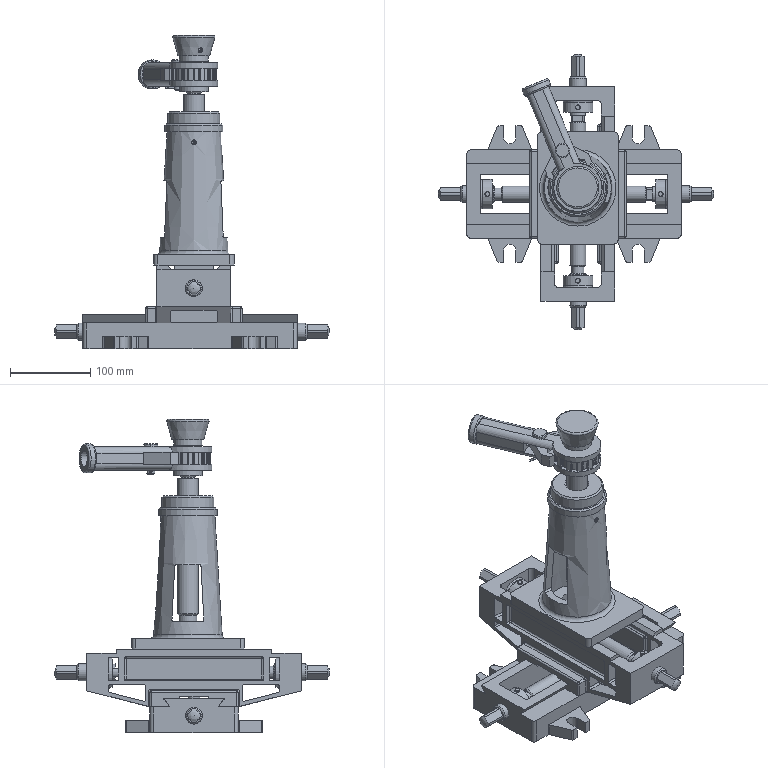Assembly | NX | mm | 32 component files | 32 solids | 906 faces | box 343 x 343 x 389.97 mm | volume 2573782 mm3 | cylinder 385 | plane 363 | cone 66 | torus 45 | sphere 40 | spline 7 | commonest cylinder face diameters 4 x153 2 x47 6 x35 10 x17 17 x16 56 x12 50 x12 21 x12
Bill of materials:
unnamed part 1 | 4 |  | Plain solid cylindrical pin with a chamfer at both ends.
unnamed part 2 | 1 |  | Prismatic block with a cross-section shaped like a rectangle with four chamfered corners (an elongated octagon). A single round through-bore runs the full length.
unnamed part 3 | 4 |  | Thick cylindrical ring or collar with a large central bore and one small radial cross-hole through the wall.
unnamed part 4 | 2 |  | Stepped cylindrical pin. A large-diameter body with a straight slot across its end steps down through a conical shoulder to a smaller-diameter spigot.
unnamed part 5 | 1 |  | Flanged cylindrical bushing with a through-bore, a chamfered flange and end, and one small radial hole in the shank.
unnamed part 6 | 2 |  | Long stepped shaft. It has a flatted tang at each end with a cross-hole, a raised collar section, a narrow necked groove, and a long main cylindrical section.
unnamed part 7 | 1 |  | Hollow, slightly tapered tubular post standing on a rectangular base plate with rounded corners. The tube wall has a rectangular side window. Two lugs project below the base, at least one with an eye hole.
unnamed part 8 | 1 |  | Lever or fork-like part. A cylindrical rod with a collar head at one end has a cross-hole near its middle. At the other end are two parallel flat plates (tines), each ending in a round eye. One eye bore has a keyway-like notch.
unnamed part 9 | 1 |  | Block with rounded edges and a cross-shaped outline in one view. A large round through-bore runs horizontally, a cylindrical boss sits on top, and side ridges or tongues run along its length.
unnamed part 10 | 1 |  | Open rectangular frame or housing with a central cavity, internal longitudinal ribs or rails, end walls with round holes, side flanges, and a tapered underside with a dovetail-like channel.
unnamed part 11 | 1 |  | Annular washer-like disc with a flat underside and a domed (curved or conical) upper face, plus a large central hole.
unnamed part 12 | 1 |  | Toothed ring with 12 evenly spaced, round-cornered rectangular teeth around the outside and a central bore with one keyway notch.
unnamed part 13 | 1 |  | Long stepped cylindrical shaft. A thin raised collar sits near one end, then a larger stepped section, then a small end spigot with a cross hole. The opposite end has a short reduced-diameter step.
unnamed part 14 | 1 |  | Pin bent from wire of roughly half-round section: a closed eye loop at one end and two parallel legs ending in angled tips, one leg slightly shorter.
unnamed part 15 | 1 |  | Flat plate of constant thickness with an irregular, roughly fan-shaped polygon outline. A large concave circular-arc cutout runs along one side, and there is one round through-hole.
unnamed part 16 | 2 |  | Cylindrical part with a slotted clevis-style fork at one end, a cross hole through both fork tines, and a stepped reduced end. The reduced end has flats forming a square-like cross-section and a domed tip.
unnamed part 17 | 1 |  | Solid block shaped like an extruded obround (stadium): two flat parallel faces, two semicircular ends and lightly rounded edges.
unnamed part 18 | 1 |  | Pin with a cylindrical shank and an enlarged head. The head has a short cylindrical band and ends in a conical point; the shank end is slightly rounded.
unnamed part 19 | 1 |  | Truncated-cone body (frustum) with a flat wide face, a rounded rim on that face, and one small radial hole through the side wall near the narrow end.
unnamed part 20 | 1 |  | Headed cylindrical pin: a short wide disc head with a chamfered edge, a plain shank, a cross hole near the free end, and a chamfered tip.
unnamed part 21 | 1 |  | Helical coil of round-section wire with open pitch along most of its length. Both end coils are closed and ground flat.
unnamed part 22 | 1 |  | Rectangular frame-like block with a long rectangular through-window. It has four tapered tabs, two on each long side, each with an open U-slot. A round hole runs through each short end wall, and a raised trapezoidal (dovetail-like) rib runs along the top.
unnamed part 23 | 1 |  | Plain flat annular ring (washer-like): a circular disc with a concentric central through-hole and flat parallel faces.
Mates:
1. fix | Base 1 component
2. touch align | MovingTable 1 face | Base 1 face
3. center | MovingTable 1 face | MovingTable 1 face | Base 1 face | Base 1 face
4. touch align | MachineBody 1 face | MovingTable 1 face
5. parallel | MachineBody 1 face | MovingTable 1 face
6. touch align | Nut_2 1 face | MovingTable 1 face
7. touch align | Nut_2 1 face | Base 1 face
8. touch align | BearingNut 1 face | MachineBody 1 face
9. touch align | BearingNut 1 face | MachineBody 1 face
10. touch align | LeadScrew 1 face | MachineBody 1 face
11. parallel | HandleSleeve 1 face | LeadScrew 1 face
12. concentric | LeadScrew 1 edge | HandleSleeve 1 edge
13. parallel | Ratchet 1 face | HandleSleeve 1 face
14. concentric | Ratchet 1 arc | HandleSleeve 1 edge
15. concentric | SphericalWasher2 1 edge | SphericalWasher 1 edge
16. concentric | SphericalWasher2 1 edge | LeadScrew 1 edge
17. touch align | TopBlock 1 face | LeadScrew 1 face
18. touch align | TopBlock 1 face | LeadScrew 1 face
19. touch align | SPRING_CYLINDER_COMPRESSION_1 1 datumaxis | HandleSleeve 1 face
20. touch align | SPRING_CYLINDER_COMPRESSION_1 1 face | HandleSleeve 1 face
21. touch align | PullPin 1 face | SPRING_CYLINDER_COMPRESSION_1 1 face
22. touch align | Pawl 1 face | HandleSleeve 1 face
23. center | Pawl 1 face | Pawl 1 face | HandleSleeve 1 face | HandleSleeve 1 face
24. touch align | Nut 1 face | MovingTable 1 face
25. parallel | Nut 1 face | MovingTable 1 face
26. touch align | HorizontalLeadScrew 2 face | MovingTable 1 face
27. touch align | Sleeve 2 face | HorizontalLeadScrew 2 face
28. touch align | Sleeve 2 face | MovingTable 1 face
29. touch align | Nut 1 face | MachineBody 1 face
30. touch align | HorizontalLeadScrew 1 face | Base 1 face
31. touch align | Sleeve 1 face | HorizontalLeadScrew 1 face
32. touch align | Sleeve 1 face | Base 1 face
33. touch align | GB_T_75_1985_SlottedSetScrew_M6x14 2 face | TopBlock 1 face
34. touch align | GB_T_75_1985_SlottedSetScrew_M6x14 1 face | MachineBody 1 face
35. concentric | GB_T_882_2008_Pin_A_Type_10x35 1 edge | HandleSleeve 1 edge
36. parallel | GB_T_91_2000_CotterPin_3_2x20 1 edge | HandleSleeve 1 face
37. concentric | GB_T_1096_2003_Key_A_6x6x14 1 edge | LeadScrew 1 edge
38. parallel | GB_T_1096_2003_Key_A_6x6x14 1 face | LeadScrew 1 face
39. touch align | GB_T_119_1_2000_CylindricalPin_6x40 4 face | Sleeve 1 face
40. center | GB_T_119_1_2000_CylindricalPin_6x40 4 face | GB_T_119_1_2000_CylindricalPin_6x40 4 face | HorizontalLeadScrew 1 face | HorizontalLeadScrew 1 face
41. touch align | GB_T_119_1_2000_CylindricalPin_6x40 3 face | HorizontalLeadScrew 1 face
42. center | GB_T_119_1_2000_CylindricalPin_6x40 3 face | GB_T_119_1_2000_CylindricalPin_6x40 3 face | HorizontalLeadScrew 1 face | HorizontalLeadScrew 1 face
43. touch align | GB_T_119_1_2000_CylindricalPin_6x40 2 face | Sleeve 2 face
44. center | GB_T_119_1_2000_CylindricalPin_6x40 2 face | GB_T_119_1_2000_CylindricalPin_6x40 2 face | HorizontalLeadScrew 2 face | HorizontalLeadScrew 2 face
45. touch align | GB_T_119_1_2000_CylindricalPin_6x40 1 face | HorizontalLeadScrew 2 face
46. center | GB_T_119_1_2000_CylindricalPin_6x40 1 face | GB_T_119_1_2000_CylindricalPin_6x40 1 face | HorizontalLeadScrew 2 face | HorizontalLeadScrew 2 face
47. concentric | RetainingRing 4 edge | MovingTable 1 edge
48. touch align | GB_T_119_1_2000_CylindricalPin_6x40 1 face | RetainingRing 4 face
49. concentric | RetainingRing 3 edge | MovingTable 1 edge
50. touch align | GB_T_119_1_2000_CylindricalPin_6x40 2 face | RetainingRing 3 face
51. concentric | RetainingRing 2 edge | Base 1 edge
52. touch align | RetainingRing 2 face | GB_T_119_1_2000_CylindricalPin_6x40 4 face
53. concentric | RetainingRing 1 edge | Base 1 edge
54. touch align | RetainingRing 1 face | GB_T_119_1_2000_CylindricalPin_6x40 3 face
55. distance | GB_T_91_2000_CotterPin_3_2x20 1 face | GB_T_882_2008_Pin_A_Type_10x35 1 face